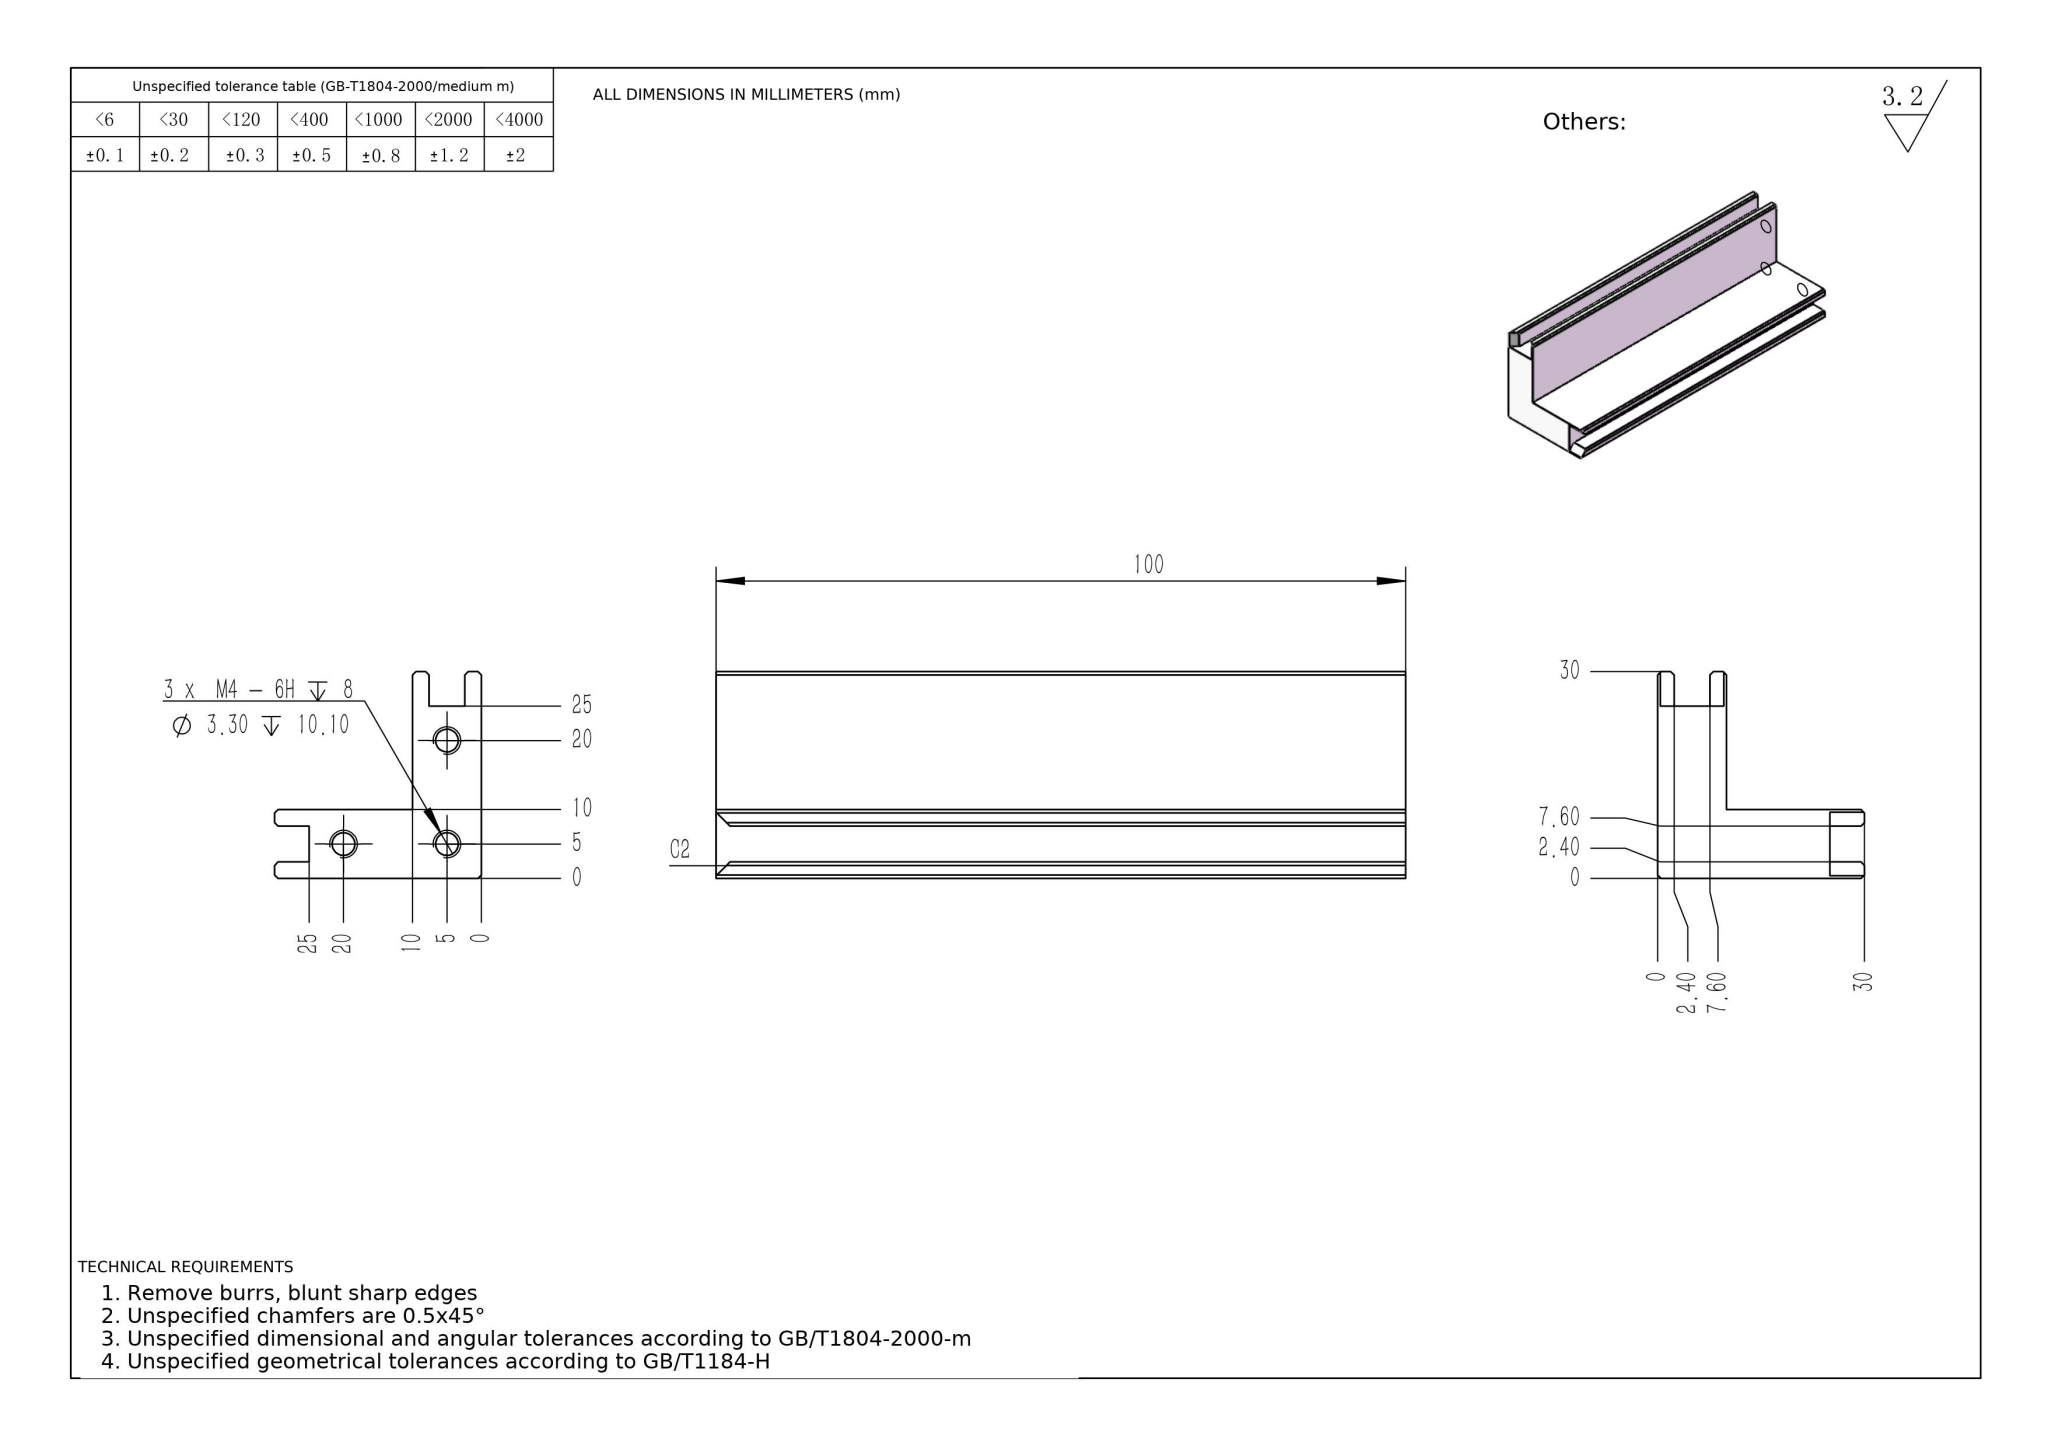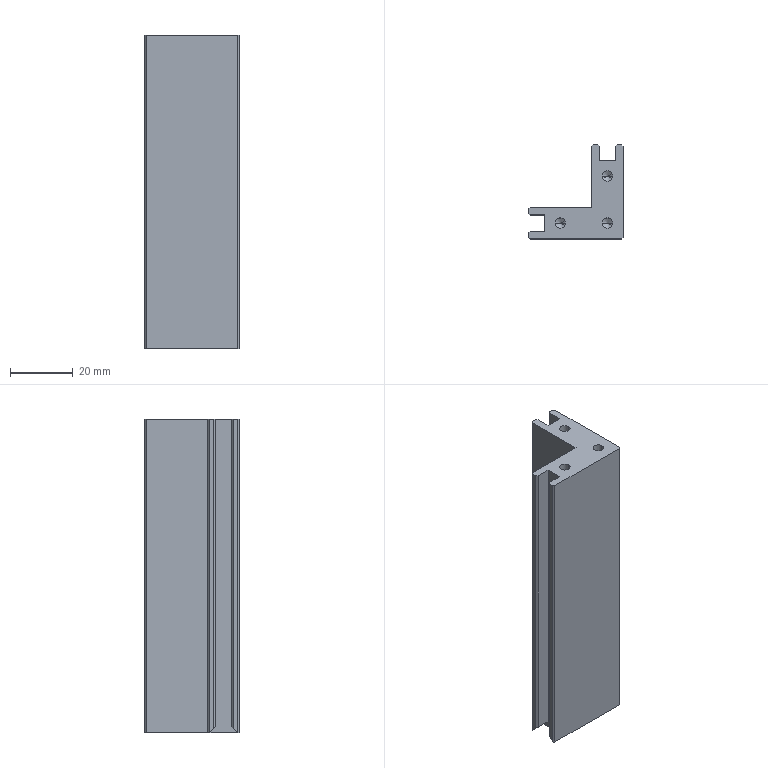Part | NX | mm | 1 solid | 41 faces | box 30 x 30 x 100 mm | volume 44381 mm3 | plane 29 | cylinder 6 | cone 6 | commonest cylinder face diameters 3.3 x6